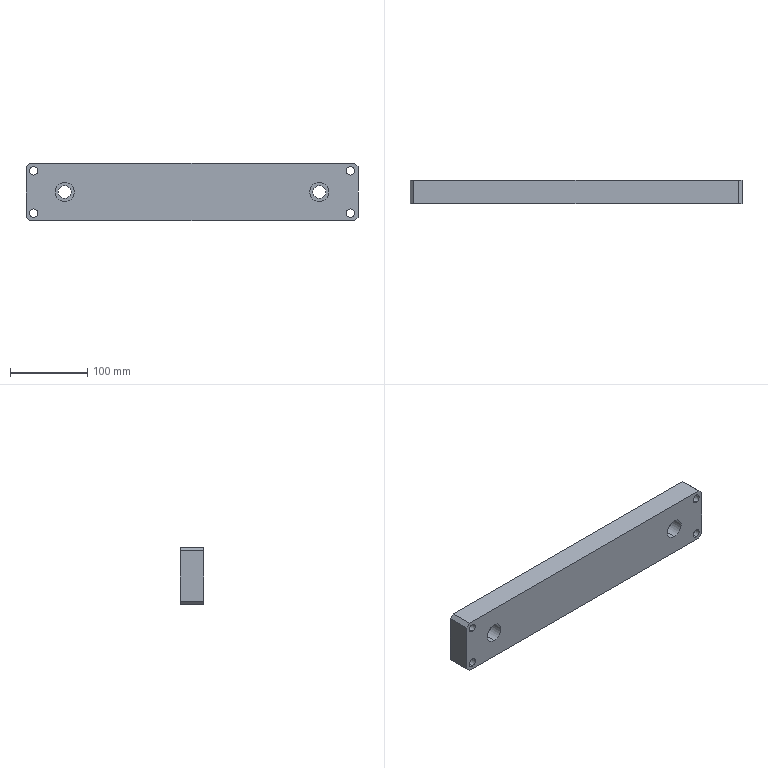Component | SolidWorks | TractionMachineBottomPlate-1 | 1 solid | 50 faces | box 430 x 30 x 75 mm | volume 918740 mm3 | cylinder 28 | plane 14 | cone 8 | commonest cylinder face diameters 11 x8 8.5 x4 25 x4 4.2 x4 40 x4 17 x4
build123d program:
from build123d import *

# Parameters (mm, degrees)
SKETCH1_W                      = 430
SKETCH1_H                      = 30
BOSS_EXTRUDE1_DEPTH            = 37.5
SKETCH2_R                      = 20
CUT_EXTRUDE1_DEPTH             = 221.298
F_11_0_11_DIAMETER_HOLE1_D     = 11
F_11_0_11_DIAMETER_HOLE1_DEPTH = 36.25
F_11_0_11_DIAMETER_HOLE1_TIP   = 3.305
M5_TAPPED_HOLE1_D              = 4.2
M5_TAPPED_HOLE1_DEPTH          = 12.4
M5_TAPPED_HOLE1_TIP            = 1.262
BOSS_EXTRUDE2_START            = -25
SKETCH7_R                      = 20
SKETCH7_R_2                    = 8.5
BOSS_EXTRUDE2_DEPTH            = 25
SKETCH8_R                      = 12.5
CUT_EXTRUDE2_DEPTH             = 16.5
M10_TAPPED_HOLE1_D             = 8.5
M10_TAPPED_HOLE1_DEPTH         = 24.5
M10_TAPPED_HOLE1_TIP           = 2.554
CHAMFER1_SIZE                  = 5


with BuildPart() as part:
    # Sketch1 → Boss-Extrude1 (new, symmetric)
    with BuildSketch(Plane.XY):
        Rectangle(SKETCH1_W, SKETCH1_H)
    extrude(amount=BOSS_EXTRUDE1_DEPTH, both=True)

    # Sketch2 → Cut-Extrude1 (cut, through all)
    with BuildSketch(Plane(origin=(0, 15, 0), x_dir=(1, 0, 0), z_dir=(0, 1, 0))):
        with Locations(Location((-165, 0, 0), (0, 0, 270))):
            Circle(SKETCH2_R)
        with Locations(Location((165, 0, 0), (0, 0, 270))):
            Circle(SKETCH2_R)
    extrude(amount=-CUT_EXTRUDE1_DEPTH, mode=Mode.SUBTRACT)

    # 11.0 _11_ Diameter Hole1
    with Locations(Plane(origin=(0, 15, 0), x_dir=(1, 0, 0), z_dir=(0, 1, 0))):
        with Locations((-205, 27.5), (-205, -27.5), (205, 27.5), (205, -27.5)):
            Hole(F_11_0_11_DIAMETER_HOLE1_D / 2, depth=F_11_0_11_DIAMETER_HOLE1_DEPTH)
            with Locations((0, 0, -(F_11_0_11_DIAMETER_HOLE1_DEPTH + F_11_0_11_DIAMETER_HOLE1_TIP / 2))):  # 118° drill point
                Cone(0, F_11_0_11_DIAMETER_HOLE1_D / 2, F_11_0_11_DIAMETER_HOLE1_TIP, mode=Mode.SUBTRACT)

    # M5 Tapped Hole1
    with Locations(Plane(origin=(0, 15, 0), x_dir=(1, 0, 0), z_dir=(0, 1, 0))):
        with Locations((40, 0), (-40, 0)):
            Hole(M5_TAPPED_HOLE1_D / 2, depth=M5_TAPPED_HOLE1_DEPTH)
            with Locations((0, 0, -(M5_TAPPED_HOLE1_DEPTH + M5_TAPPED_HOLE1_TIP / 2))):  # 118° drill point
                Cone(0, M5_TAPPED_HOLE1_D / 2, M5_TAPPED_HOLE1_TIP, mode=Mode.SUBTRACT)

    # Sketch7 → Boss-Extrude2 (add)
    with BuildSketch(Plane.XZ.offset(15).offset(BOSS_EXTRUDE2_START)):
        with Locations(Location((-165, 0, 0), (0, 0, 90))):
            Circle(SKETCH7_R)
        with Locations(Location((-165, 0, 0), (0, 0, 270))):
            Circle(SKETCH7_R_2, mode=Mode.SUBTRACT)
    boss_extrude2 = extrude(amount=BOSS_EXTRUDE2_DEPTH)

    # Sketch8 → Cut-Extrude2 (cut)
    with BuildSketch(Plane.XZ.offset(15)):
        with Locations(Location((-165, 0, 0), (0, 0, 270))):
            Circle(SKETCH8_R)
    cut_extrude2 = extrude(amount=-CUT_EXTRUDE2_DEPTH, mode=Mode.SUBTRACT)

    # Mirror1: Boss-Extrude2, Cut-Extrude2 across plane
    add(boss_extrude2.mirror(Plane(origin=(0, 0, 0), x_dir=(0, 0, 1), z_dir=(1, 0, 0))))
    add(cut_extrude2.mirror(Plane(origin=(0, 0, 0), x_dir=(0, 0, 1), z_dir=(1, 0, 0))), mode=Mode.SUBTRACT)

    # M10 Tapped Hole1
    with Locations(Plane(origin=(0, 0, -37.5), x_dir=(-1, 0, 0), z_dir=(0, 0, -1))):
        with Locations((-27.5, 0), (27.5, 0)):
            Hole(M10_TAPPED_HOLE1_D / 2, depth=M10_TAPPED_HOLE1_DEPTH)
            with Locations((0, 0, -(M10_TAPPED_HOLE1_DEPTH + M10_TAPPED_HOLE1_TIP / 2))):  # 118° drill point
                Cone(0, M10_TAPPED_HOLE1_D / 2, M10_TAPPED_HOLE1_TIP, mode=Mode.SUBTRACT)

    # Chamfer1
    chamfer1_edges = [part.edges().sort_by_distance(p)[0] for p in [
        (-215, 0, 37.5),
        (215, 0, 37.5),
        (-215, 0, -37.5),
        (215, 0, -37.5),
    ]]
    chamfer(chamfer1_edges, length=CHAMFER1_SIZE)


solid = part.part

# Placed as in the assembly
solid = solid.moved(Location((-29.507, -304.411, 458), (0, 0, 0)))